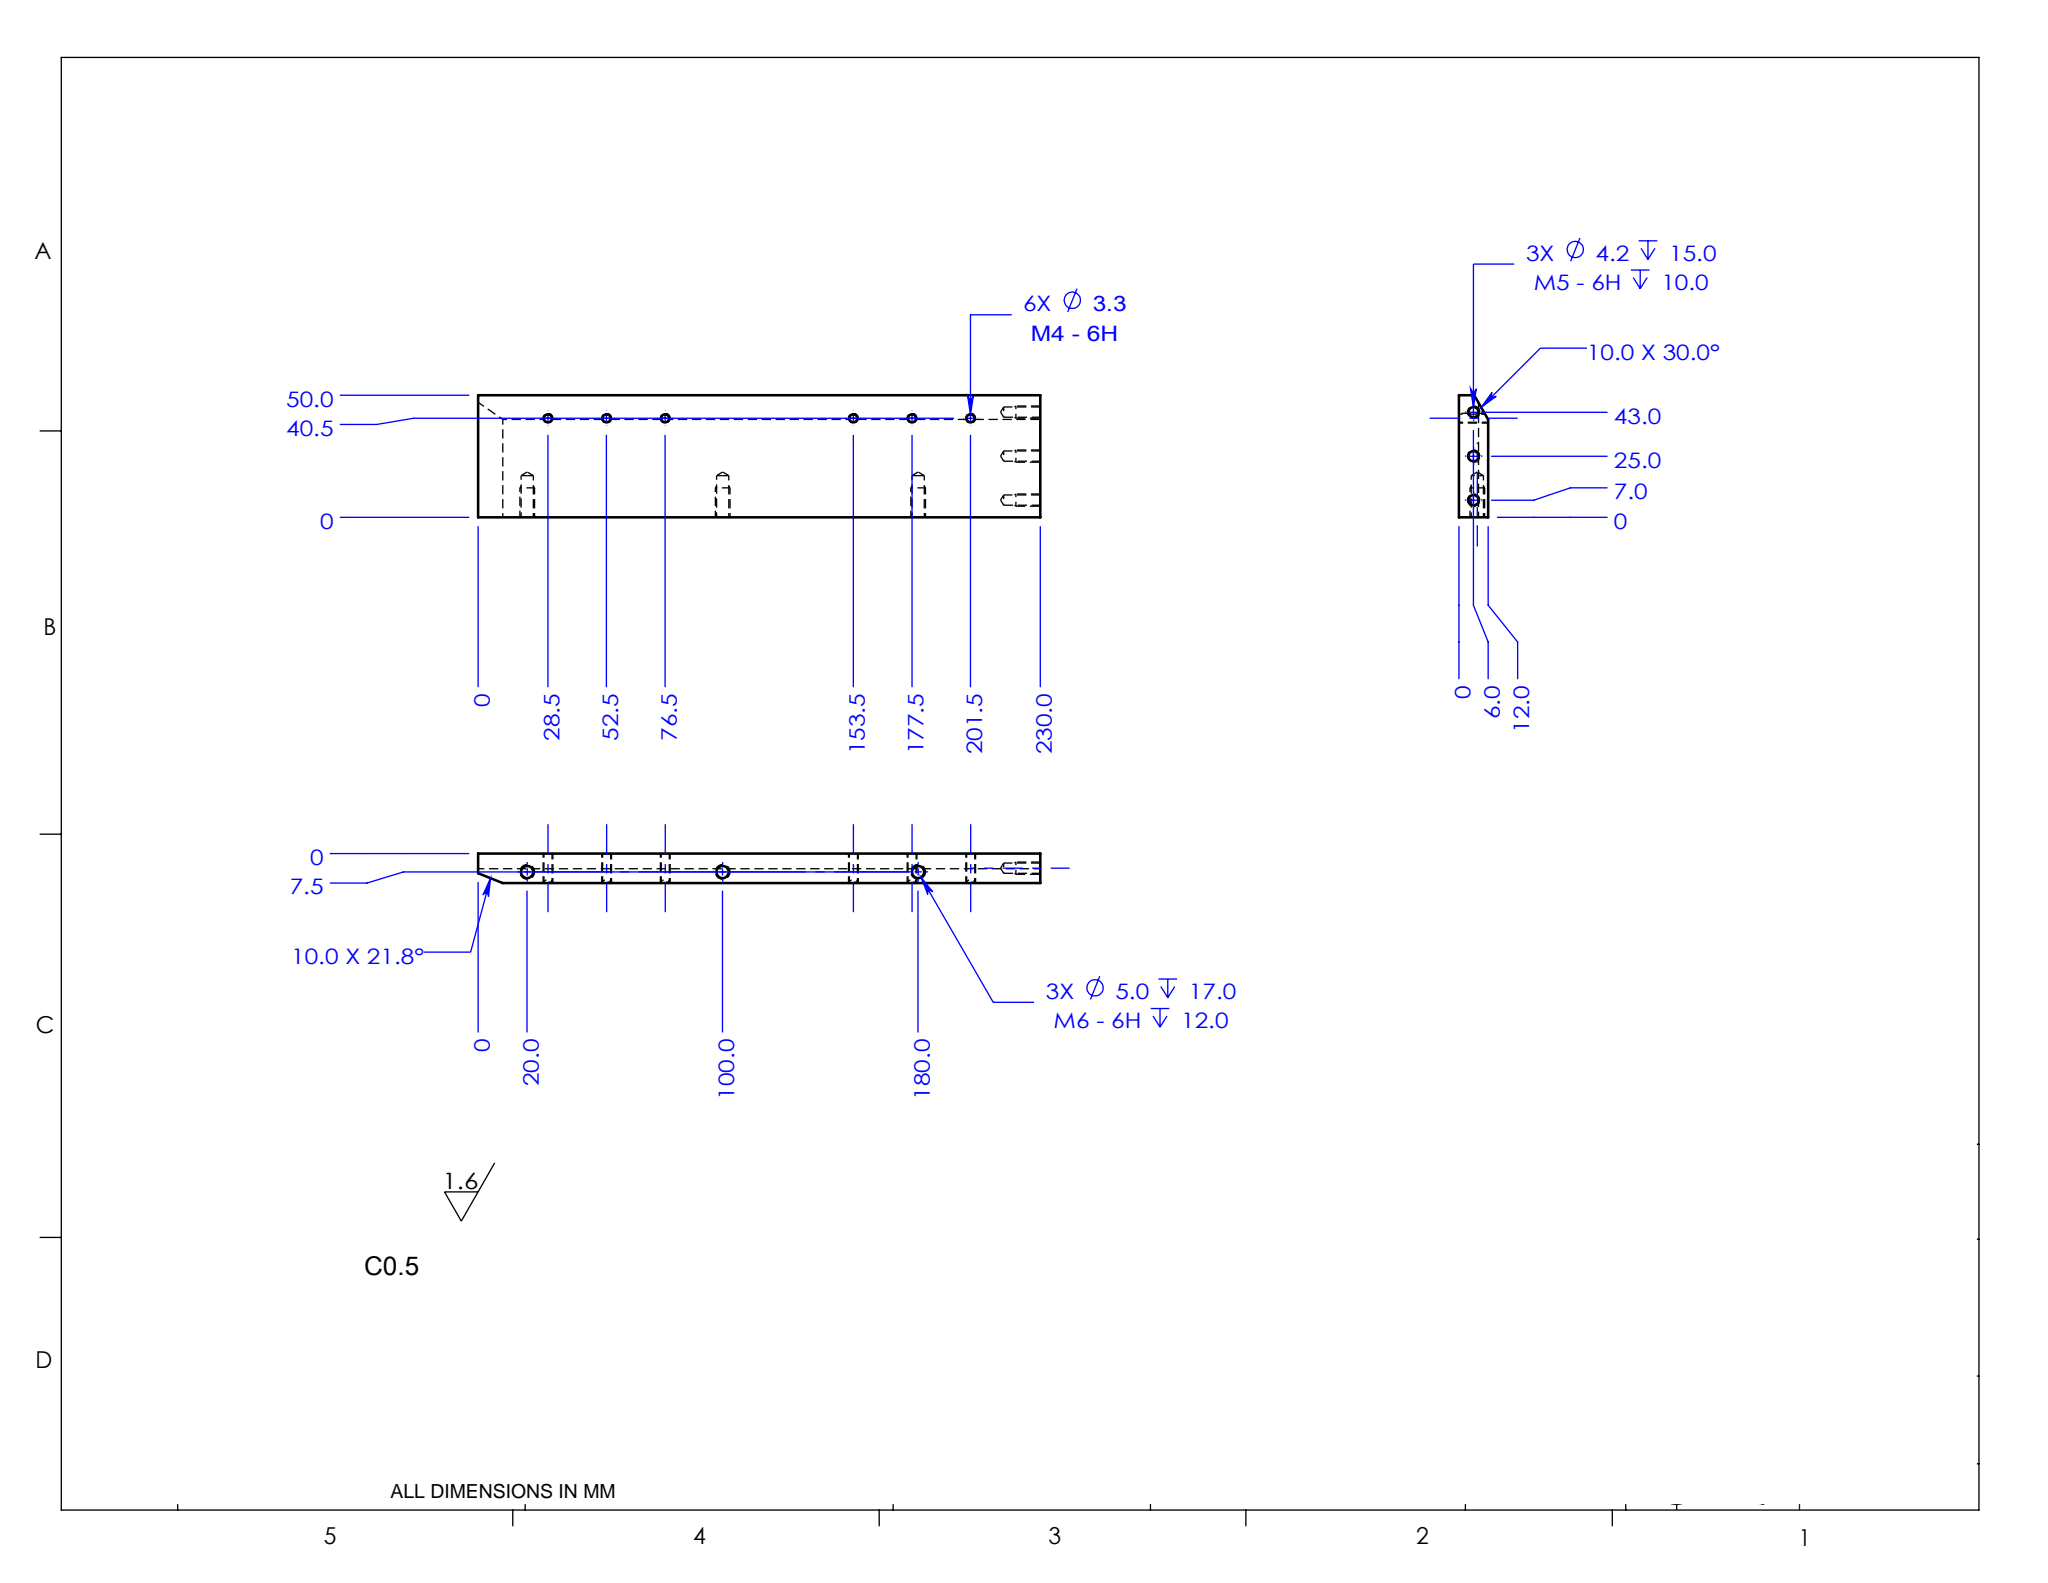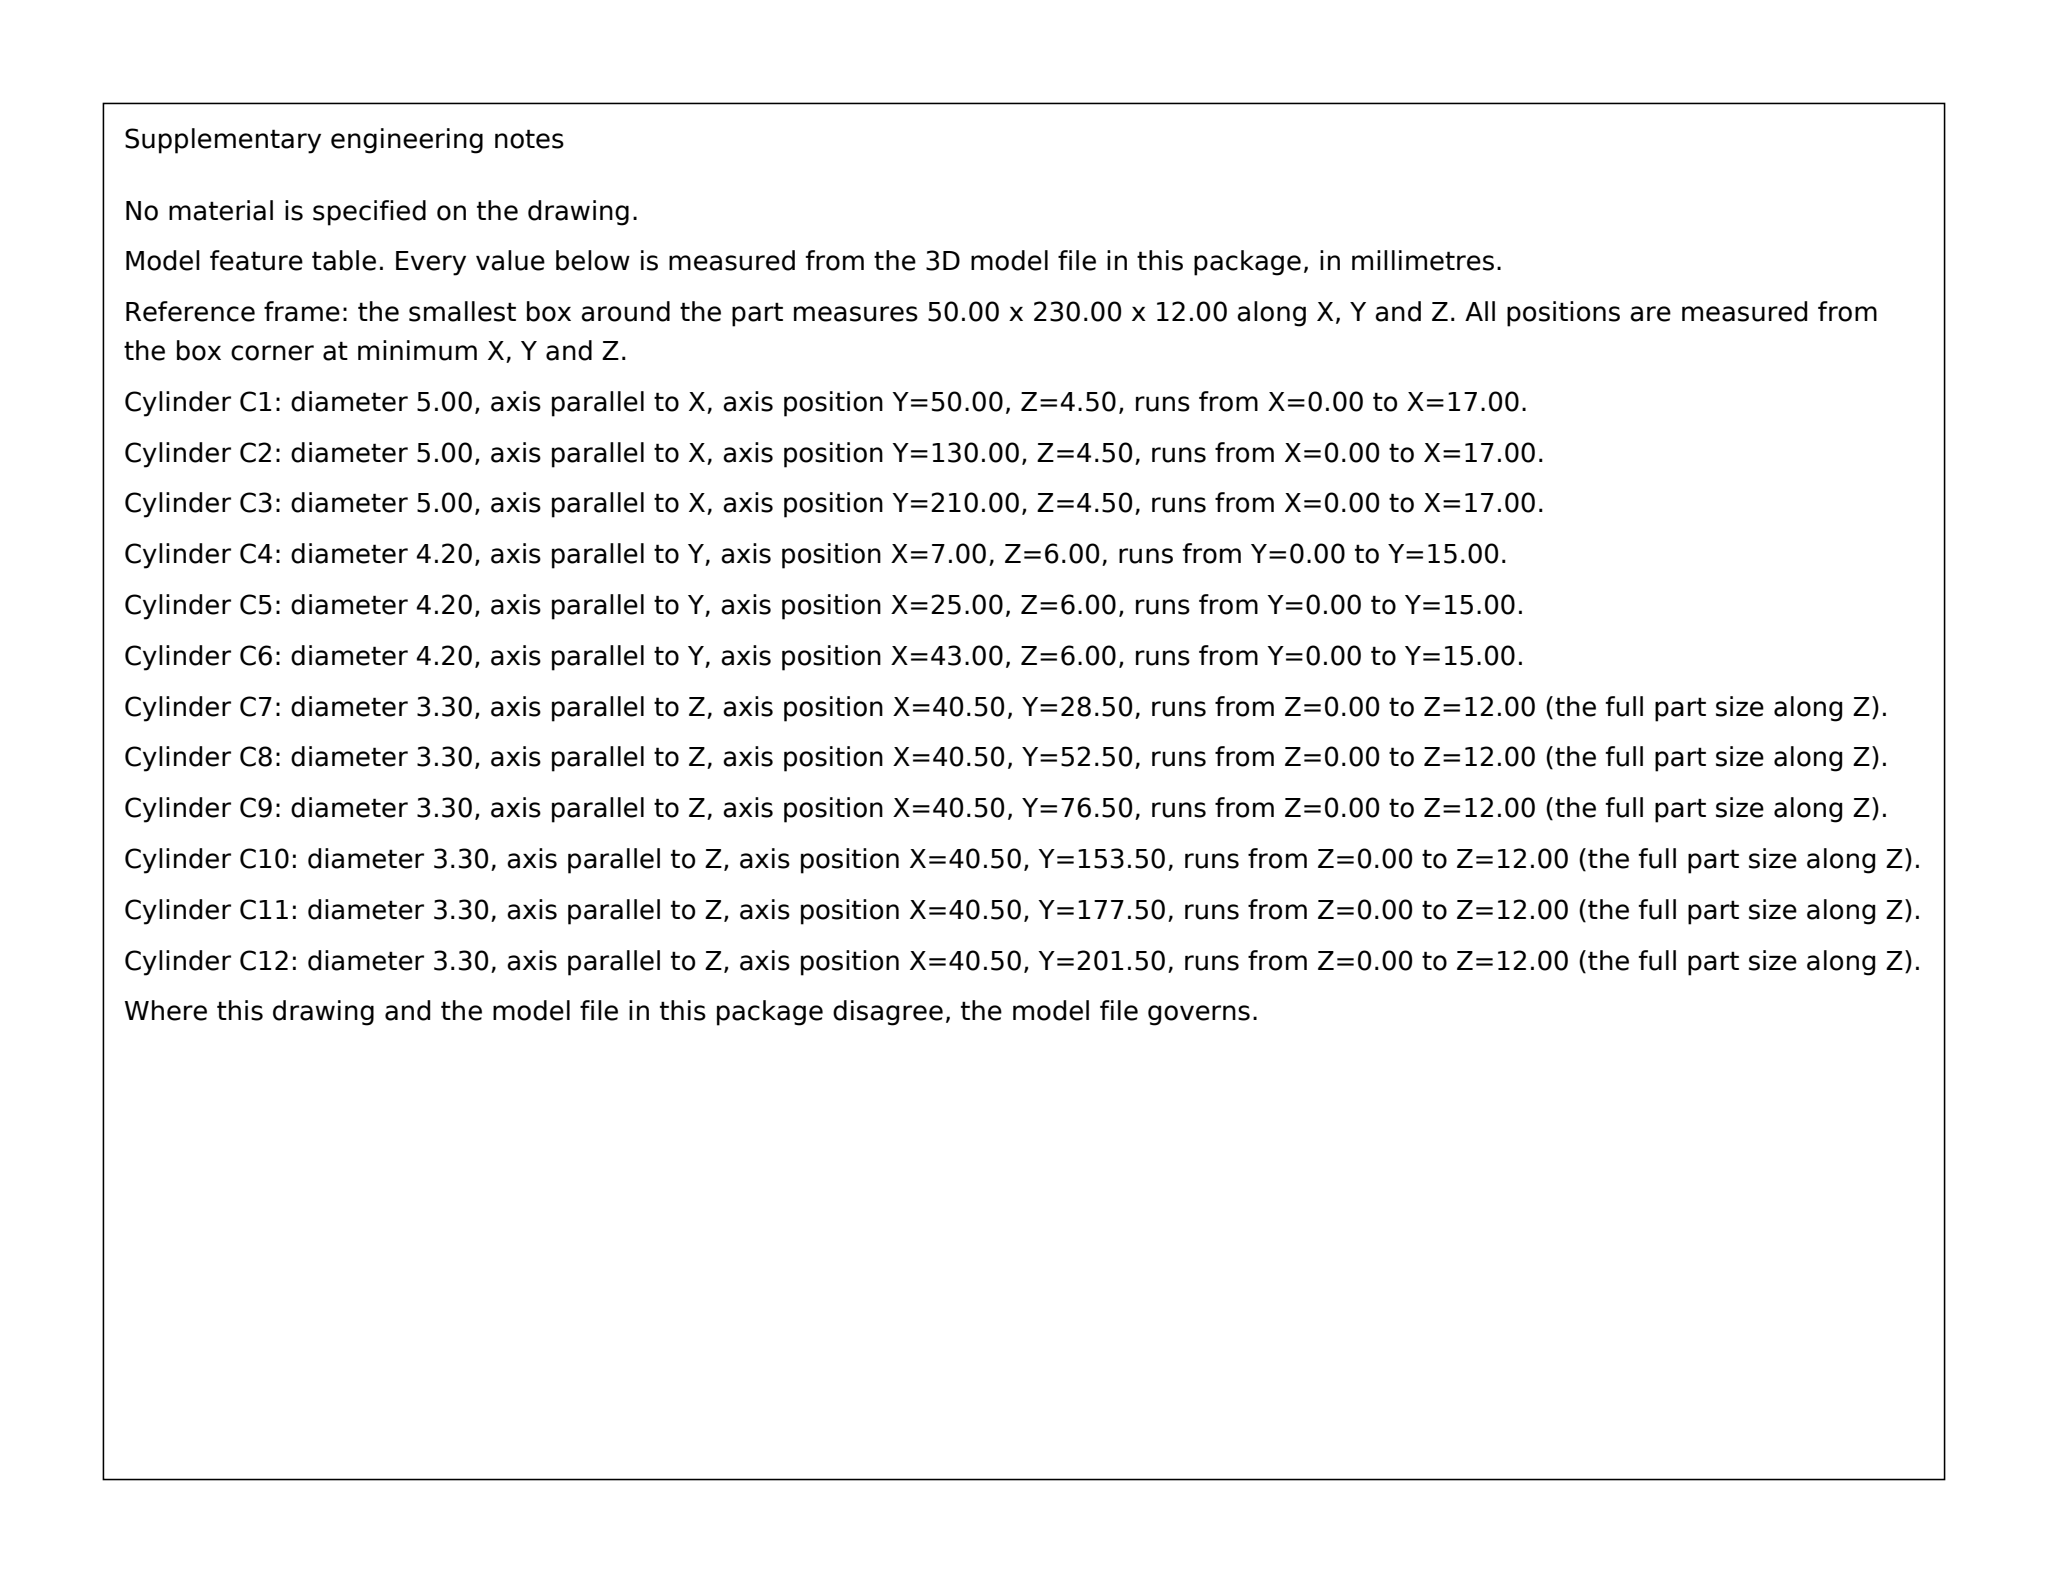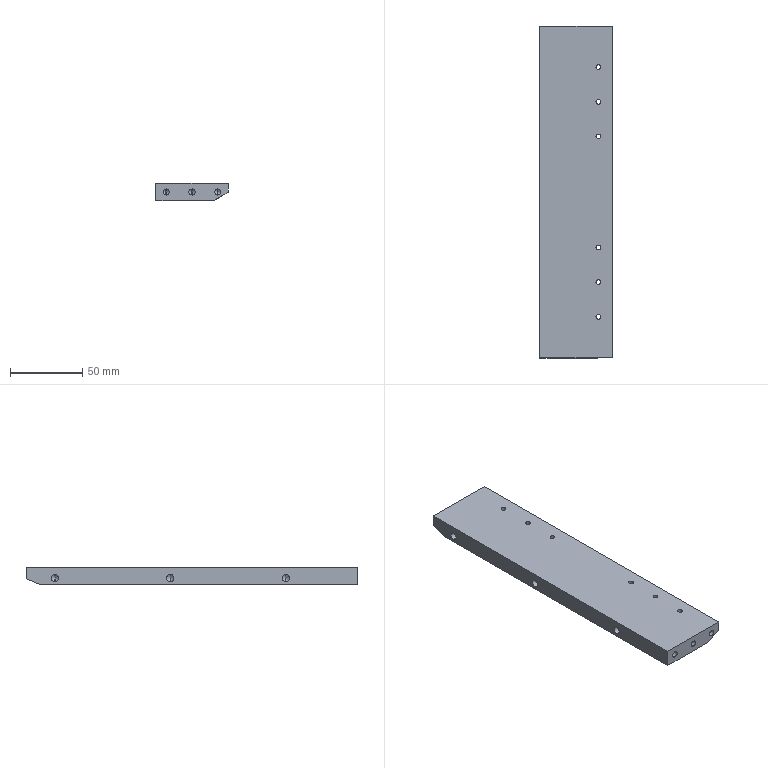Part | SolidWorks | mm | 1 solid | 44 faces | box 50 x 230 x 12 mm | volume 128246 mm3 | cylinder 24 | cone 12 | plane 8 | commonest cylinder face diameters 3.3 x12 4.2 x6 5 x6